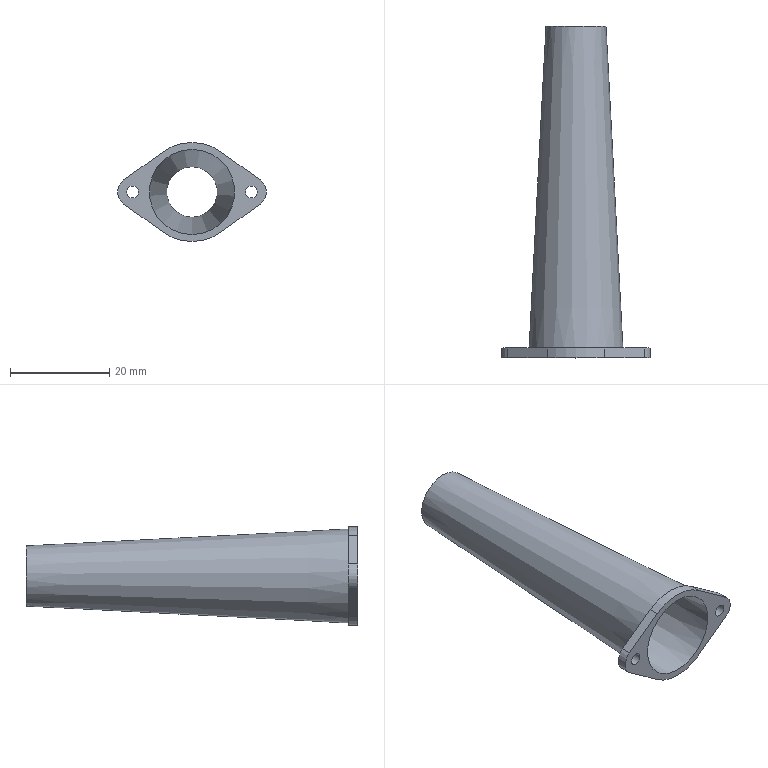Component | NX | 7 | 1 solid | 15 faces | volume 3296 mm3 | plane 7 | cylinder 6 | cone 2 | commonest cylinder face diameters 6 x2 20 x2 2.4 x2